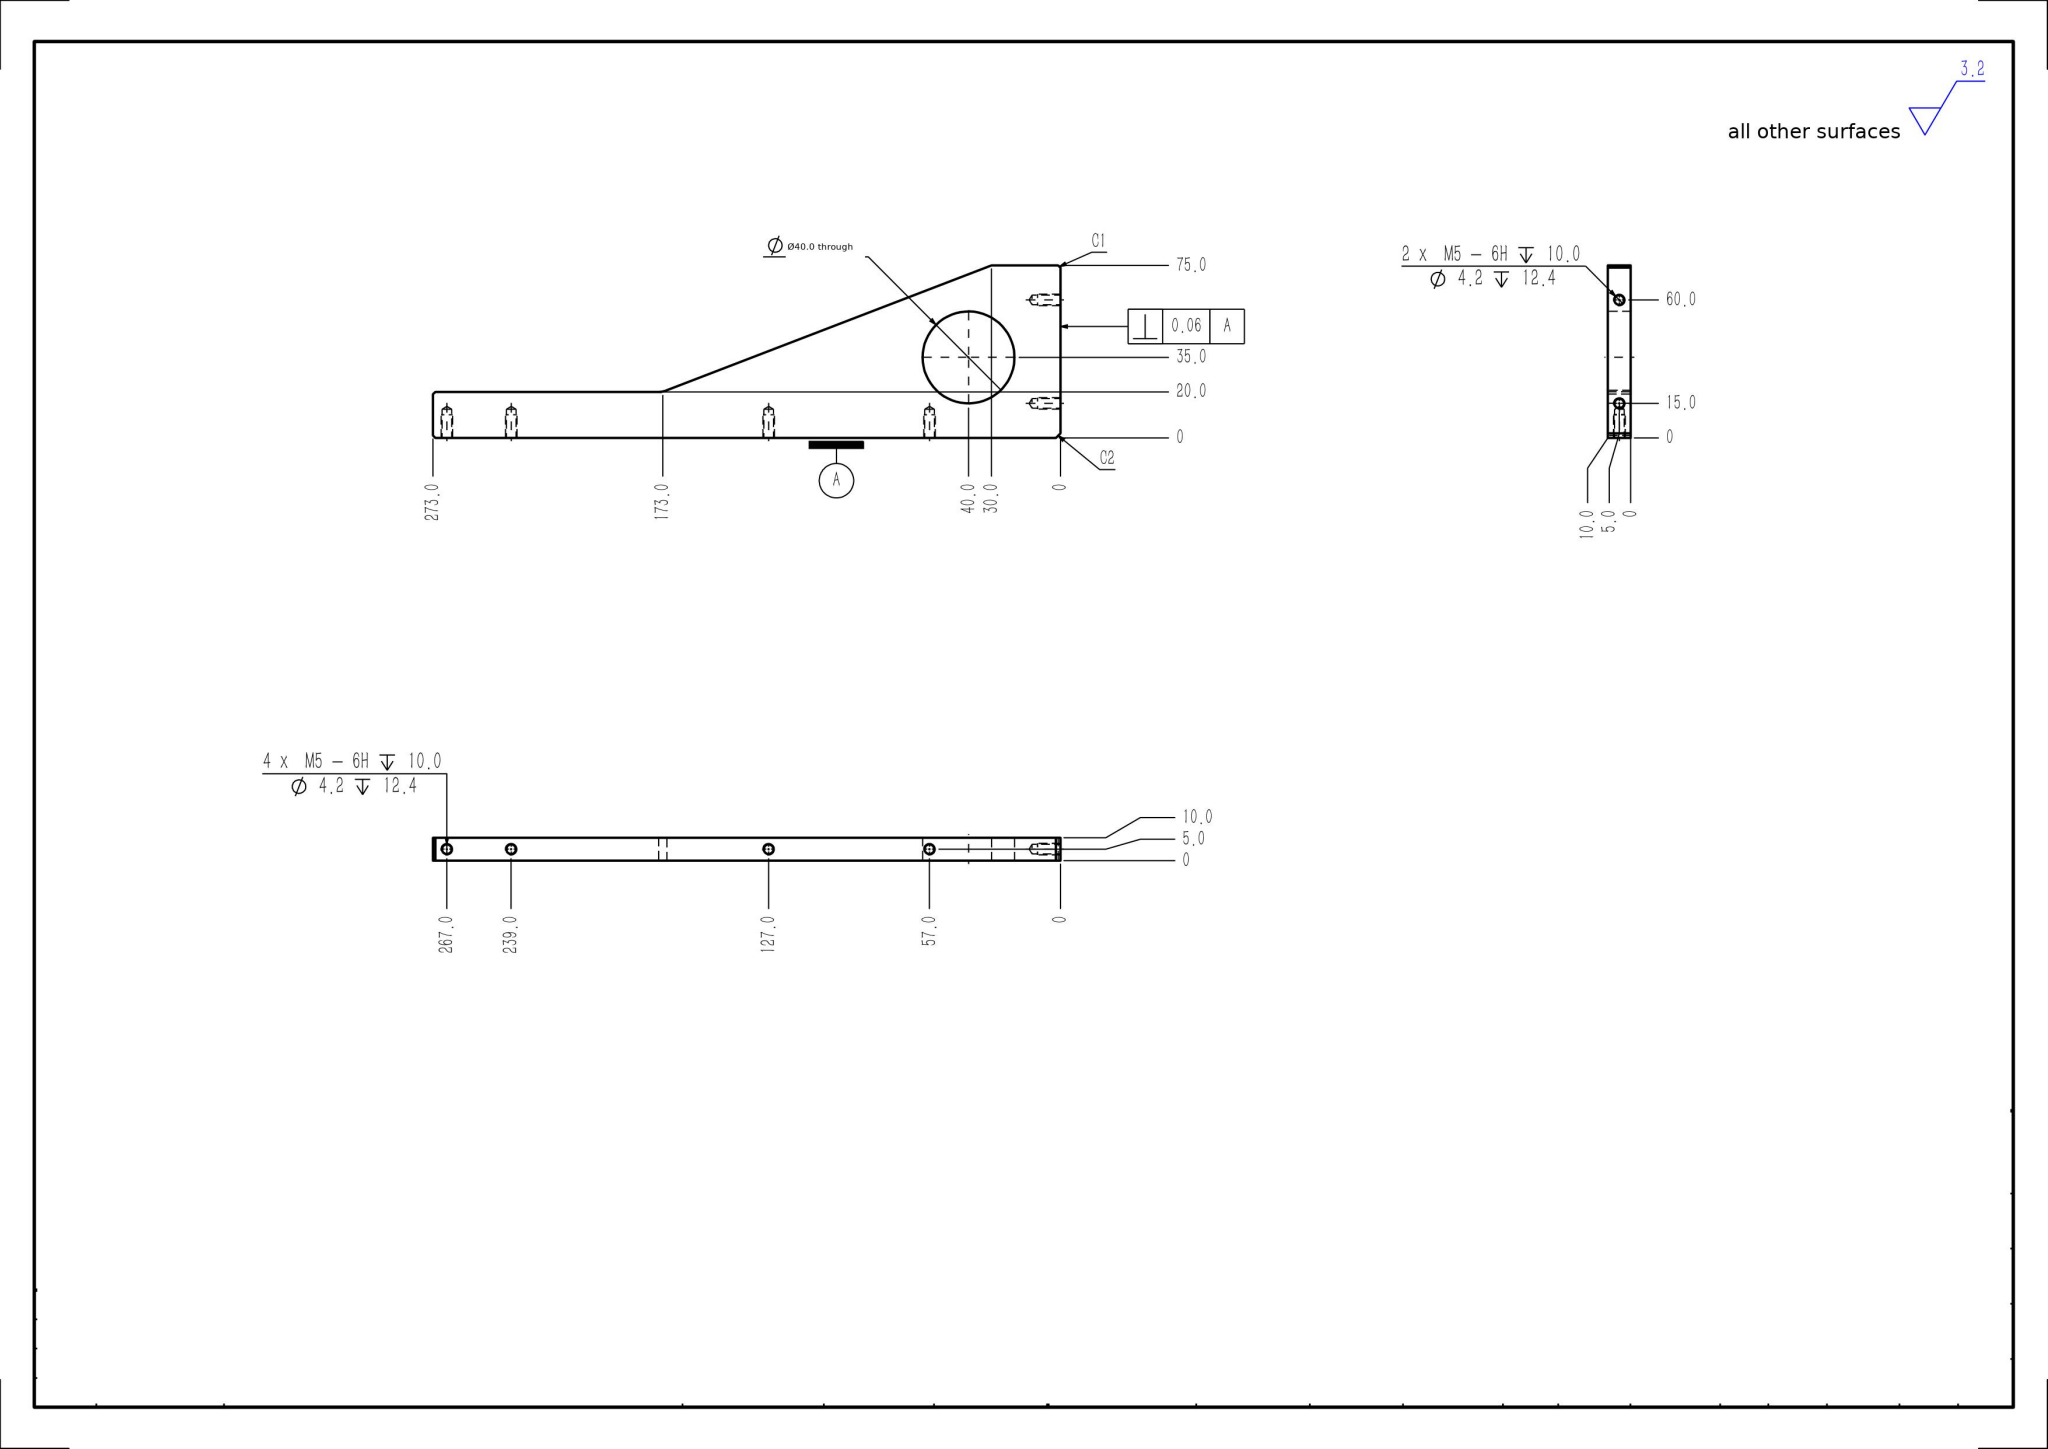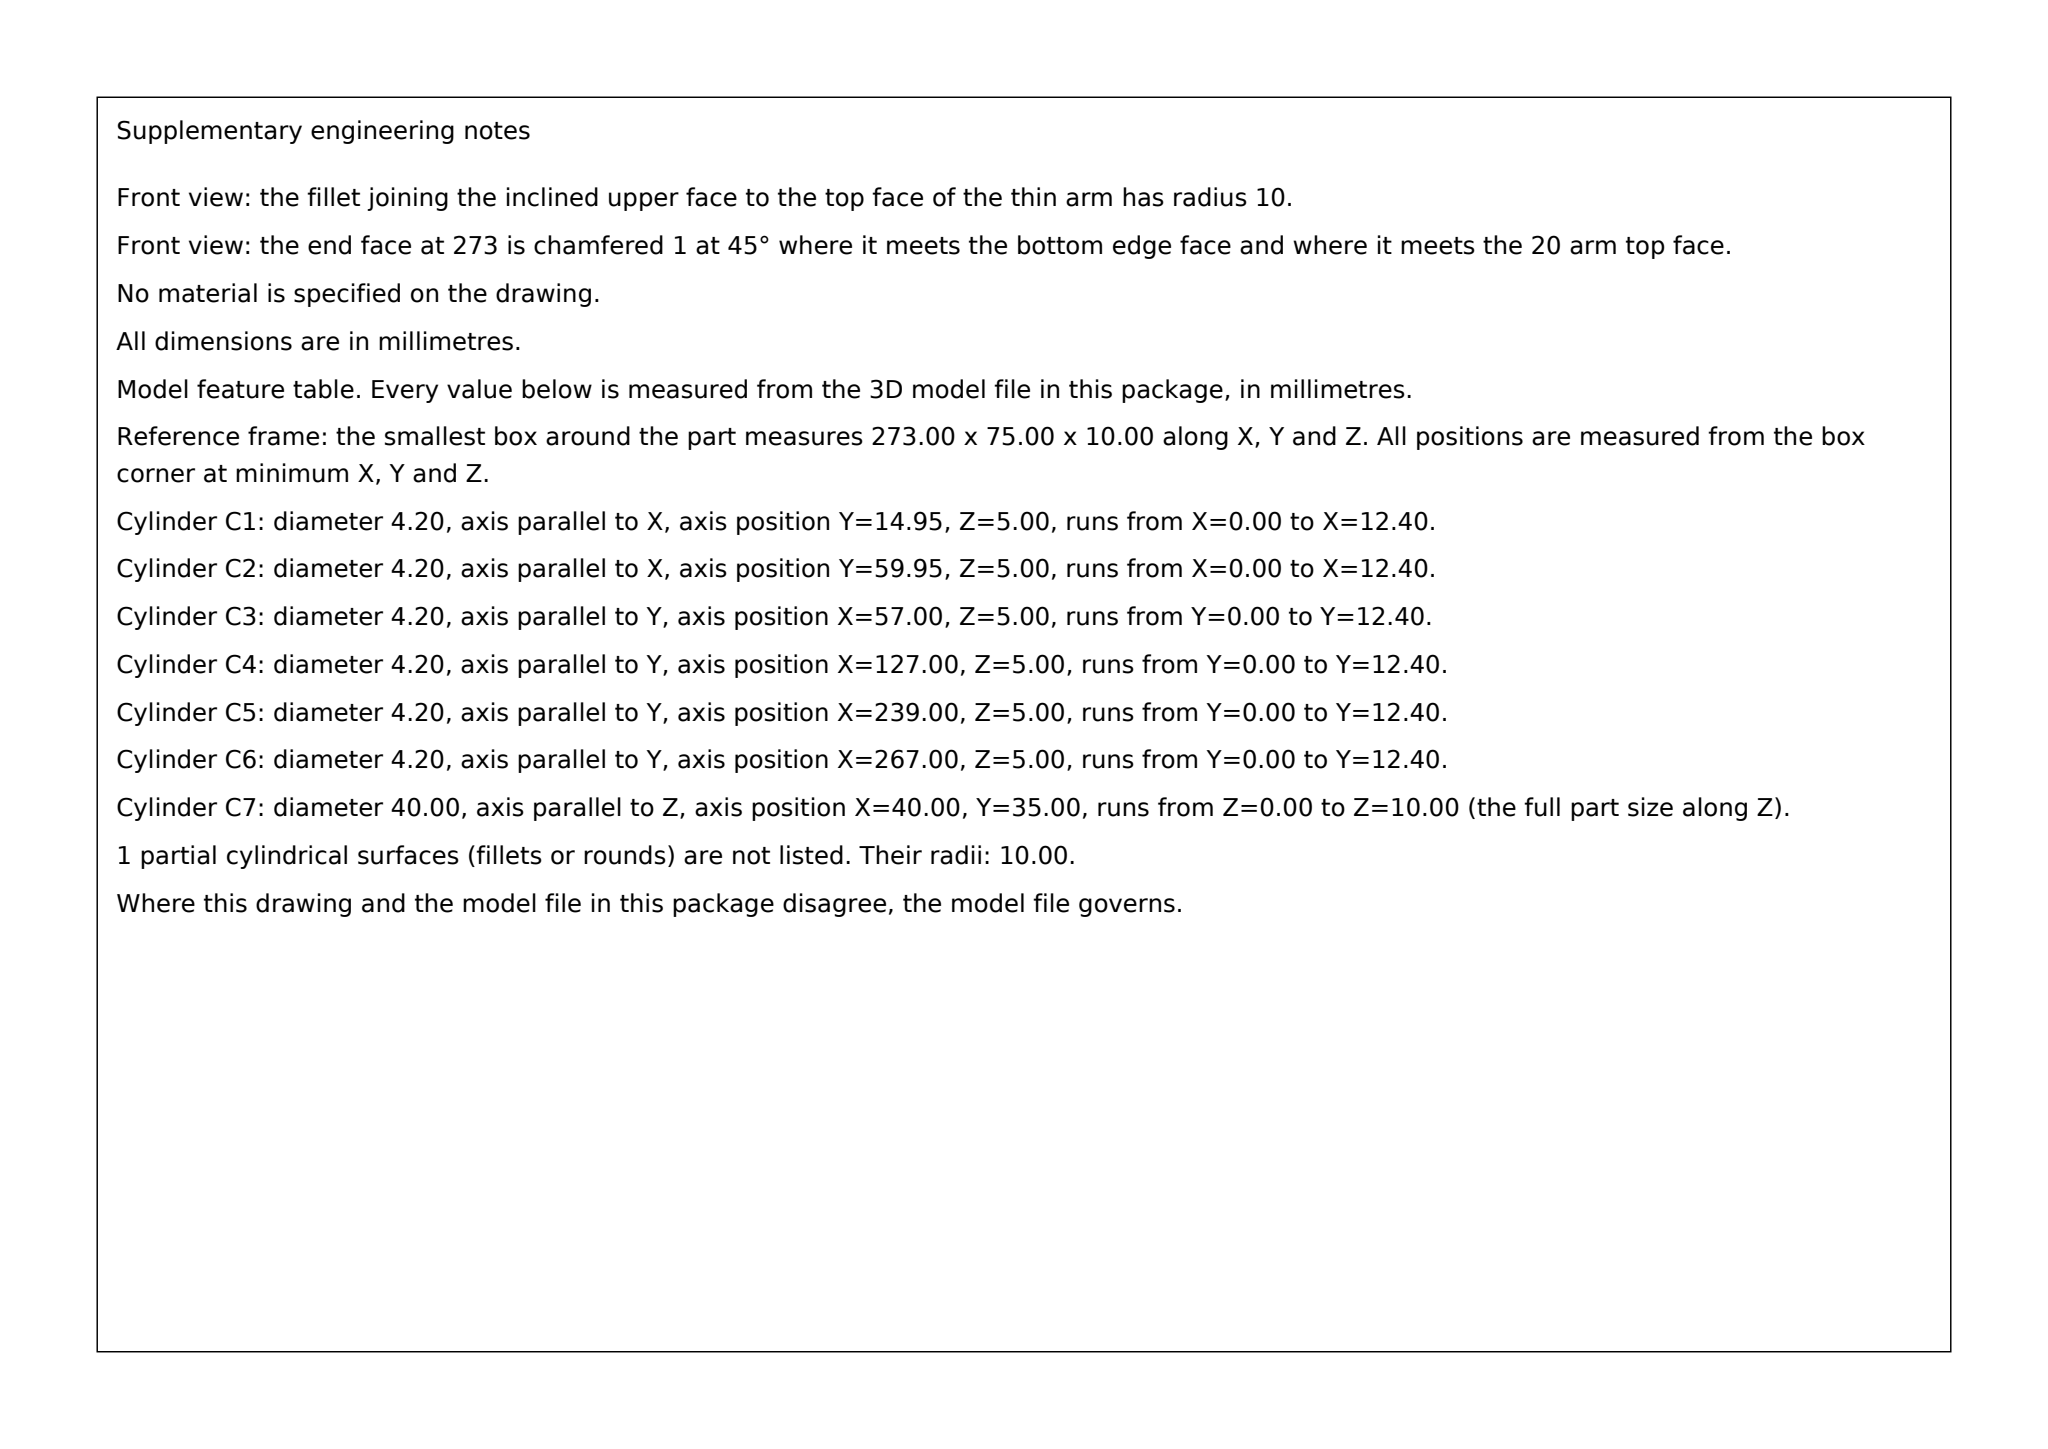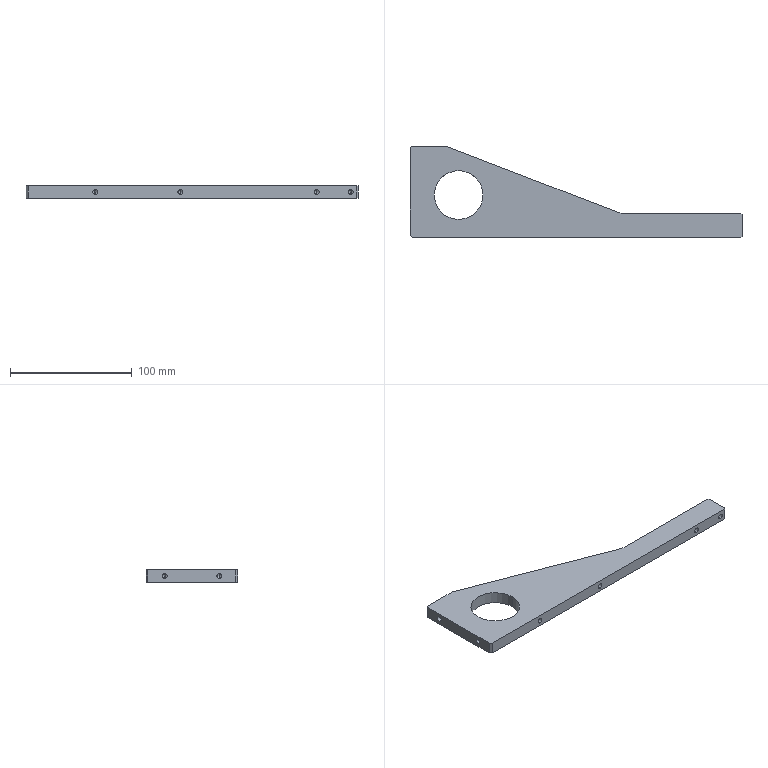Part | SolidWorks | mm | 1 solid | 39 faces | box 273 x 75 x 10 mm | volume 96760 mm3 | cylinder 15 | cone 12 | plane 12 | commonest cylinder face diameters 4.2 x12 40 x2 20 x1
Drawing notes:
2X C1 CHAMFER AT 273.0 END (BOTH EDGES) | from the solid: bbox_xyz x=273.0 end face; planes x=0.0 and x=273.0 define 273 long bar; 2 chamfered edges at far end
R10.0 FILLET AT STEP, TANGENT AT 173.0 | from the solid: cylinder [20.0,'z',[174.86,30.0],10.0] = R10.0 vertical blend at step, full 10 thk; tangent point at X=173.0 from 0 datum
build123d program:
from build123d import *

# Parameters (mm, degrees)
SKETCH1_W             = 273
SKETCH1_H             = 75
BOSS_EXTRUDE1_DEPTH   = 10
SKETCH2_W             = 100
SKETCH2_H             = 55
CUT_EXTRUDE1_DEPTH    = 142.91
CUT_EXTRUDE2_DEPTH    = 142.91
M5_TAPPED_HOLE1_D     = 4.2
M5_TAPPED_HOLE1_DEPTH = 12.4
M5_TAPPED_HOLE1_TIP   = 1.262
M5_TAPPED_HOLE2_D     = 4.2
M5_TAPPED_HOLE2_DEPTH = 12.4
M5_TAPPED_HOLE2_TIP   = 1.262
CHAMFER1_SIZE         = 1
CHAMFER2_SIZE         = 2
FILLET1_R             = 10
SKETCH8_R             = 20
CUT_EXTRUDE3_DEPTH    = 142.91


with BuildPart() as part:
    # Sketch1 → Boss-Extrude1 (new body)
    with BuildSketch(Plane.XY):
        Rectangle(SKETCH1_W, SKETCH1_H)
    extrude(amount=BOSS_EXTRUDE1_DEPTH)

    # Sketch2 → Cut-Extrude1 (cut, through all)
    with BuildSketch(Plane.XY.offset(10)):
        with Locations((86.5, 10)):
            Rectangle(SKETCH2_W, SKETCH2_H)
    extrude(amount=-CUT_EXTRUDE1_DEPTH, mode=Mode.SUBTRACT)

    # Sketch3 → Cut-Extrude2 (cut, through all)
    with BuildSketch(Plane(origin=(0, 0, 0), x_dir=(-1, 0, 0), z_dir=(0, 0, -1))):
        Polygon((-36.5, -17.5), (106.5, 37.5), (-36.5, 37.5), align=None)
    extrude(amount=-CUT_EXTRUDE2_DEPTH, mode=Mode.SUBTRACT)

    # M5 Tapped Hole1
    with Locations(Plane(origin=(0, -37.5, 0), x_dir=(-1, 0, 0), z_dir=(0, -1, 0))):
        with Locations((79.5, -5), (-130.5, -5), (-102.5, -5), (9.5, -5)):
            Hole(M5_TAPPED_HOLE1_D / 2, depth=M5_TAPPED_HOLE1_DEPTH)
            with Locations((0, 0, -(M5_TAPPED_HOLE1_DEPTH + M5_TAPPED_HOLE1_TIP / 2))):  # 118° drill point
                Cone(0, M5_TAPPED_HOLE1_D / 2, M5_TAPPED_HOLE1_TIP, mode=Mode.SUBTRACT)

    # M5 Tapped Hole2
    with Locations(Plane.ZY.offset(136.5)):
        with Locations((5, 22.45), (5, -22.55)):
            Hole(M5_TAPPED_HOLE2_D / 2, depth=M5_TAPPED_HOLE2_DEPTH)
            with Locations((0, 0, -(M5_TAPPED_HOLE2_DEPTH + M5_TAPPED_HOLE2_TIP / 2))):  # 118° drill point
                Cone(0, M5_TAPPED_HOLE2_D / 2, M5_TAPPED_HOLE2_TIP, mode=Mode.SUBTRACT)

    # Chamfer1
    chamfer1_edges = [part.edges().sort_by_distance(p)[0] for p in [
        (136.5, -17.5, 5),
        (-136.5, 37.5, 5),
        (136.5, -37.5, 5),
    ]]
    chamfer(chamfer1_edges, length=CHAMFER1_SIZE)

    # Chamfer2
    chamfer2_edges = [part.edges().sort_by_distance(p)[0] for p in [
        (-136.5, -37.5, 5),
    ]]
    chamfer(chamfer2_edges, length=CHAMFER2_SIZE)

    # Fillet1
    fillet1_edges = [part.edges().sort_by_distance(p)[0] for p in [
        (36.5, -17.5, 5),
    ]]
    fillet(fillet1_edges, radius=FILLET1_R)

    # Sketch8 → Cut-Extrude3 (cut, through all)
    with BuildSketch(Plane.XY.offset(10)):
        with Locations((-96.5, -2.5)):
            Circle(SKETCH8_R)
    extrude(amount=-CUT_EXTRUDE3_DEPTH, mode=Mode.SUBTRACT)


solid = part.part